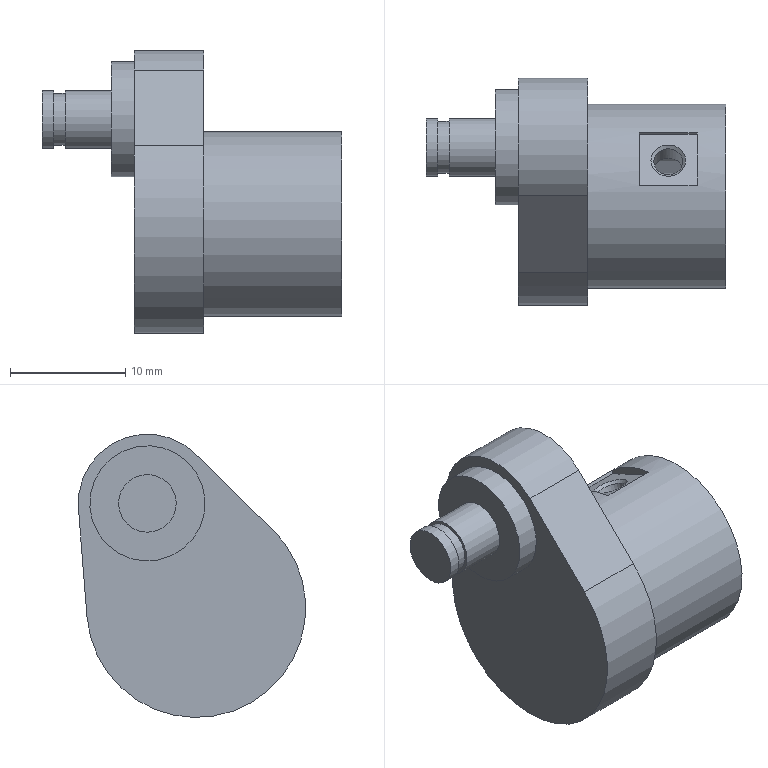Component | NX | CRANK | 1 solid | 26 faces | volume 3893 mm3 | plane 15 | cylinder 9 | cone 1 | spline 1 | commonest cylinder face diameters 10 x2 5 x2 16 x1 19 x1 12 x1 4.5 x1 2.5 x1